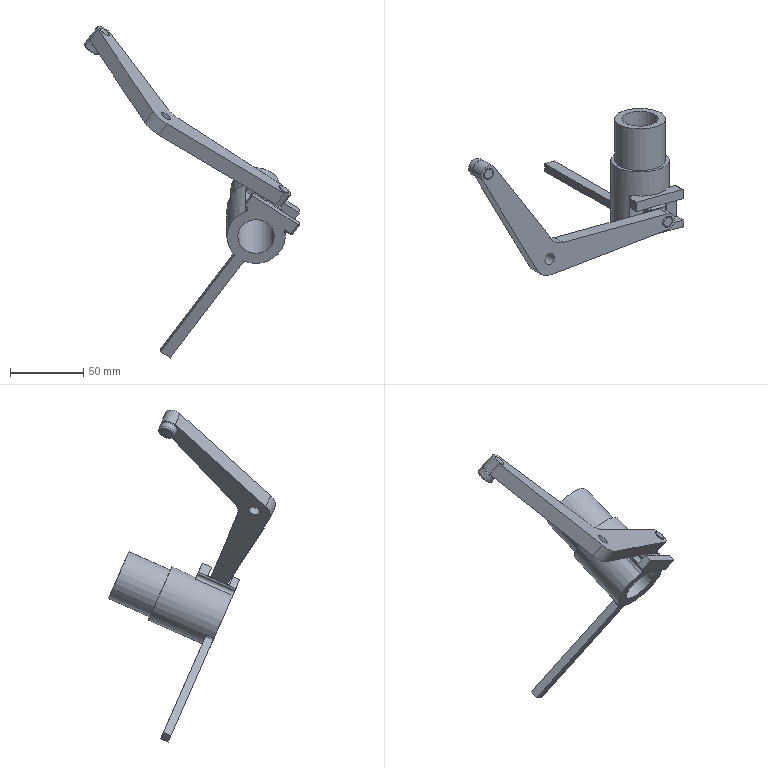Assembly | NX | mm | 6 component files | 6 solids | 87 faces | volume 91931 mm3 | cylinder 36 | plane 35 | sphere 10 | cone 4 | torus 2 | commonest cylinder face diameters 4 x13 2 x8 8 x7 24 x2 40 x1 35 x1 25 x1 12 x1
Bill of materials:
unnamed part 1 | 1 |  | Short thick-walled ring or sleeve: a cylinder with a through bore along its axis and rounded or chamfered outer edges on both end faces.
unnamed part 2 | 1 |  | Solid round cylinder or pin with flat end faces and a small chamfer or edge break at both ends.
unnamed part 3 | 1 |  | Flat bent plate link: an L- or V-shaped bar of constant thickness with rounded ends and three through holes, one at each arm end and one near the inside of the bend.
unnamed part 4 | 1 |  | Rectangular or square block with heavily rounded edges and corners and one round through hole running between two opposite faces.
unnamed part 5 | 1 |  | Solid round cylinder or pin with flat end faces and a small chamfer or edge break at both ends.
unnamed part 6 | 1 |  | Stepped hollow cylindrical body (two outer diameters, through bore) with a slim straight rectangular strip extending outward from near its base, and a rectangular slotted or H-shaped tab block on the side of the larger-diameter section.
Mates:
1. touch align | qu_bing 1 edge | xuan_zhuan_zhou 1 edge
2. touch align | hua_kuai 1 face | zhou_pei 1 face
3. touch align | hua_kuai 1 face | zhou_pei 1 face
4. touch align | hua_kuai 1 edge | xuan_zhuan_zhou 1 edge
5. touch align | yuan_huan_kuai 1 face | xuanzhuan_1 1 edge
6. touch align | yuan_huan_kuai 1 face | xuanzhuan_1 1 face
7. touch align | xuanzhuan_1 1 face | qu_bing 1 face
8. touch align | xuanzhuan_1 1 edge | qu_bing 1 edge